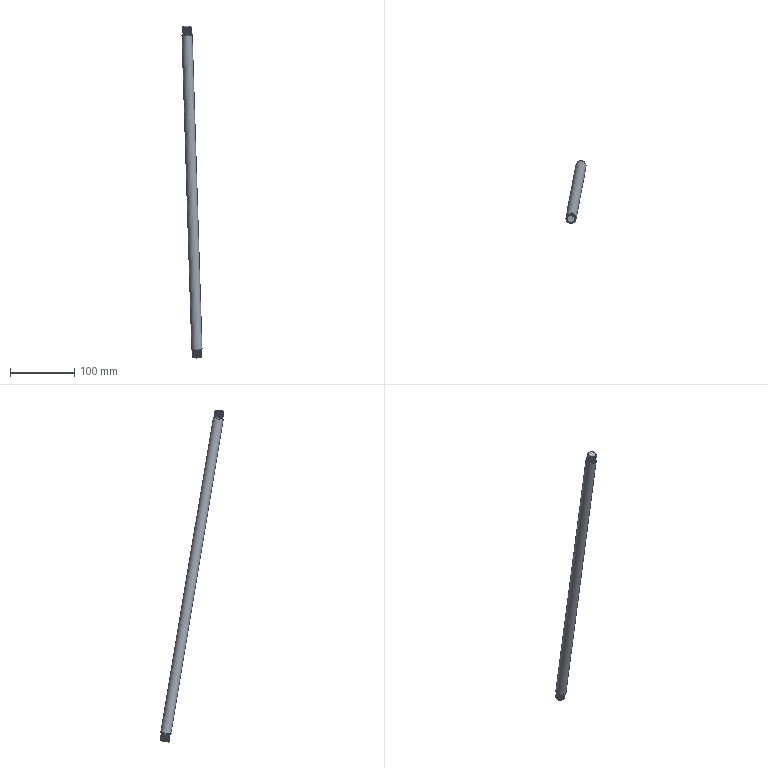Component | NX | CONTROL_ROD | 1 solid | 24 faces | volume 103432 mm3 | plane 7 | cylinder 7 | spline 6 | cone 4 | commonest cylinder face diameters 14 x2 12 x2 10 x1 16 x1 11 x1